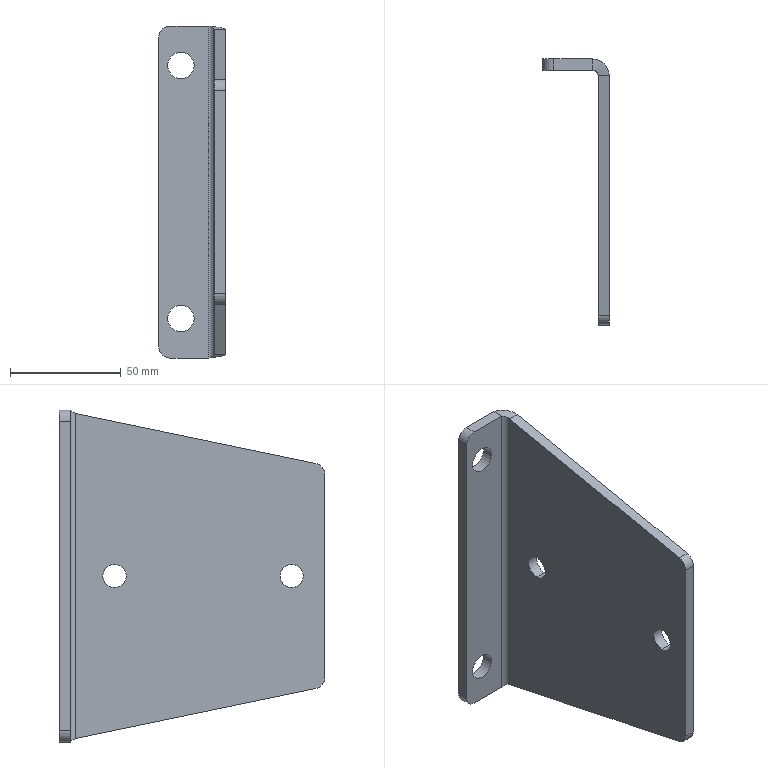Component | SolidWorks | JGS01-0001EndCorner-1 | 1 solid | 26 faces | box 30 x 120 x 150 mm | volume 90055 mm3 | cylinder 14 | plane 10 | spline 2 | commonest cylinder face diameters 10.5 x4 12 x4 10 x4 15 x1 5 x1 | material Plain Carbon Steel
STEP:
#1=COLOUR_RGB('',0.7922,0.8196,0.9333);
#2=FILL_AREA_STYLE_COLOUR('',#1);
#3=FILL_AREA_STYLE('',(#2));
#4=SURFACE_STYLE_FILL_AREA(#3);
#5=SURFACE_SIDE_STYLE('',(#4));
#6=SURFACE_STYLE_USAGE(.BOTH.,#5);
#7=PRESENTATION_STYLE_ASSIGNMENT((#6));
#8=CARTESIAN_POINT('',(-6.855,0.3688,13.707));
#9=VERTEX_POINT('',#8);
#10=CARTESIAN_POINT('',(-6.855,0.3688,13.293));
#11=VERTEX_POINT('',#10);
#12=CARTESIAN_POINT('',(-6.855,0.3688,13.5));
#13=DIRECTION('',(1.,0.,0.));
#14=DIRECTION('',(0.,0.,-1.));
#15=AXIS2_PLACEMENT_3D('',#12,#13,#14);
#16=CIRCLE('',#15,0.2067);
#17=EDGE_CURVE('',#9,#11,#16,.T.);
#18=ORIENTED_EDGE('',*,*,#17,.F.);
#19=CARTESIAN_POINT('',(-6.658,0.3688,13.707));
#20=VERTEX_POINT('',#19);
#21=CARTESIAN_POINT('',(-6.855,0.3688,13.707));
#22=DIRECTION('',(1.,0.,0.));
#23=VECTOR('',#22,39.37);
#24=LINE('',#21,#23);
#25=EDGE_CURVE('',#9,#20,#24,.T.);
#26=ORIENTED_EDGE('',*,*,#25,.T.);
#27=CARTESIAN_POINT('',(-6.658,0.3688,13.293));
#28=VERTEX_POINT('',#27);
#29=CARTESIAN_POINT('',(-6.658,0.3688,13.5));
#30=DIRECTION('',(1.,0.,0.));
#31=DIRECTION('',(0.,0.,-1.));
#32=AXIS2_PLACEMENT_3D('',#29,#30,#31);
#33=CIRCLE('',#32,0.2067);
#34=EDGE_CURVE('',#20,#28,#33,.T.);
#35=ORIENTED_EDGE('',*,*,#34,.T.);
#36=CARTESIAN_POINT('',(-6.855,0.3688,13.293));
#37=DIRECTION('',(1.,0.,0.));
#38=VECTOR('',#37,39.37);
#39=LINE('',#36,#38);
#40=EDGE_CURVE('',#11,#28,#39,.T.);
#41=ORIENTED_EDGE('',*,*,#40,.F.);
#42=EDGE_LOOP('',(#18,#26,#35,#41));
#43=FACE_OUTER_BOUND('',#42,.T.);
#44=CARTESIAN_POINT('',(-6.855,0.3688,13.5));
#45=DIRECTION('',(1.,0.,0.));
#46=DIRECTION('',(0.,0.,-1.));
#47=AXIS2_PLACEMENT_3D('',#44,#45,#46);
#48=CYLINDRICAL_SURFACE('',#47,0.2067);
#49=ADVANCED_FACE('',(#43),#48,.F.);
#50=CARTESIAN_POINT('',(-6.855,-2.781,13.707));
#51=VERTEX_POINT('',#50);
#52=CARTESIAN_POINT('',(-6.855,-2.781,13.293));
#53=VERTEX_POINT('',#52);
#54=CARTESIAN_POINT('',(-6.855,-2.781,13.5));
#55=DIRECTION('',(1.,0.,0.));
#56=DIRECTION('',(0.,0.,-1.));
#57=AXIS2_PLACEMENT_3D('',#54,#55,#56);
#58=CIRCLE('',#57,0.2067);
#59=EDGE_CURVE('',#51,#53,#58,.T.);
#60=ORIENTED_EDGE('',*,*,#59,.F.);
#61=CARTESIAN_POINT('',(-6.658,-2.781,13.707));
#62=VERTEX_POINT('',#61);
#63=CARTESIAN_POINT('',(-6.855,-2.781,13.707));
#64=DIRECTION('',(1.,0.,0.));
#65=VECTOR('',#64,39.37);
#66=LINE('',#63,#65);
#67=EDGE_CURVE('',#51,#62,#66,.T.);
#68=ORIENTED_EDGE('',*,*,#67,.T.);
#69=CARTESIAN_POINT('',(-6.658,-2.781,13.293));
#70=VERTEX_POINT('',#69);
#71=CARTESIAN_POINT('',(-6.658,-2.781,13.5));
#72=DIRECTION('',(1.,0.,0.));
#73=DIRECTION('',(0.,0.,-1.));
#74=AXIS2_PLACEMENT_3D('',#71,#72,#73);
#75=CIRCLE('',#74,0.2067);
#76=EDGE_CURVE('',#62,#70,#75,.T.);
#77=ORIENTED_EDGE('',*,*,#76,.T.);
#78=CARTESIAN_POINT('',(-6.855,-2.781,13.293));
#79=DIRECTION('',(1.,0.,0.));
#80=VECTOR('',#79,39.37);
#81=LINE('',#78,#80);
#82=EDGE_CURVE('',#53,#70,#81,.T.);
#83=ORIENTED_EDGE('',*,*,#82,.F.);
#84=EDGE_LOOP('',(#60,#68,#77,#83));
#85=FACE_OUTER_BOUND('',#84,.T.);
#86=CARTESIAN_POINT('',(-6.855,-2.781,13.5));
#87=DIRECTION('',(1.,0.,0.));
#88=DIRECTION('',(0.,0.,-1.));
#89=AXIS2_PLACEMENT_3D('',#86,#87,#88);
#90=CYLINDRICAL_SURFACE('',#89,0.2067);
#91=ADVANCED_FACE('',(#85),#90,.F.);
#92=CARTESIAN_POINT('',(-7.209,1.156,15.75));
#93=VERTEX_POINT('',#92);
#94=CARTESIAN_POINT('',(-7.682,1.156,15.75));
#95=VERTEX_POINT('',#94);
#96=CARTESIAN_POINT('',(-7.446,1.156,15.75));
#97=DIRECTION('',(0.,1.,0.));
#98=DIRECTION('',(-1.,0.,0.));
#99=AXIS2_PLACEMENT_3D('',#96,#97,#98);
#100=CIRCLE('',#99,0.2362);
#101=EDGE_CURVE('',#93,#95,#100,.T.);
#102=ORIENTED_EDGE('',*,*,#101,.F.);
#103=CARTESIAN_POINT('',(-7.209,1.353,15.75));
#104=VERTEX_POINT('',#103);
#105=CARTESIAN_POINT('',(-7.209,1.156,15.75));
#106=DIRECTION('',(0.,1.,0.));
#107=VECTOR('',#106,39.37);
#108=LINE('',#105,#107);
#109=EDGE_CURVE('',#93,#104,#108,.T.);
#110=ORIENTED_EDGE('',*,*,#109,.T.);
#111=CARTESIAN_POINT('',(-7.682,1.353,15.75));
#112=VERTEX_POINT('',#111);
#113=CARTESIAN_POINT('',(-7.446,1.353,15.75));
#114=DIRECTION('',(0.,1.,0.));
#115=DIRECTION('',(-1.,0.,0.));
#116=AXIS2_PLACEMENT_3D('',#113,#114,#115);
#117=CIRCLE('',#116,0.2362);
#118=EDGE_CURVE('',#104,#112,#117,.T.);
#119=ORIENTED_EDGE('',*,*,#118,.T.);
#120=CARTESIAN_POINT('',(-7.682,1.156,15.75));
#121=DIRECTION('',(0.,1.,0.));
#122=VECTOR('',#121,39.37);
#123=LINE('',#120,#122);
#124=EDGE_CURVE('',#95,#112,#123,.T.);
#125=ORIENTED_EDGE('',*,*,#124,.F.);
#126=EDGE_LOOP('',(#102,#110,#119,#125));
#127=FACE_OUTER_BOUND('',#126,.T.);
#128=CARTESIAN_POINT('',(-7.446,1.156,15.75));
#129=DIRECTION('',(0.,1.,0.));
#130=DIRECTION('',(-1.,0.,0.));
#131=AXIS2_PLACEMENT_3D('',#128,#129,#130);
#132=CYLINDRICAL_SURFACE('',#131,0.2362);
#133=ADVANCED_FACE('',(#127),#132,.F.);
#134=CARTESIAN_POINT('',(-7.209,1.156,11.25));
#135=VERTEX_POINT('',#134);
#136=CARTESIAN_POINT('',(-7.682,1.156,11.25));
#137=VERTEX_POINT('',#136);
#138=CARTESIAN_POINT('',(-7.446,1.156,11.25));
#139=DIRECTION('',(0.,1.,0.));
#140=DIRECTION('',(-1.,0.,0.));
#141=AXIS2_PLACEMENT_3D('',#138,#139,#140);
#142=CIRCLE('',#141,0.2362);
#143=EDGE_CURVE('',#135,#137,#142,.T.);
#144=ORIENTED_EDGE('',*,*,#143,.F.);
#145=CARTESIAN_POINT('',(-7.209,1.353,11.25));
#146=VERTEX_POINT('',#145);
#147=CARTESIAN_POINT('',(-7.209,1.156,11.25));
#148=DIRECTION('',(0.,1.,0.));
#149=VECTOR('',#148,39.37);
#150=LINE('',#147,#149);
#151=EDGE_CURVE('',#135,#146,#150,.T.);
#152=ORIENTED_EDGE('',*,*,#151,.T.);
#153=CARTESIAN_POINT('',(-7.682,1.353,11.25));
#154=VERTEX_POINT('',#153);
#155=CARTESIAN_POINT('',(-7.446,1.353,11.25));
#156=DIRECTION('',(0.,1.,0.));
#157=DIRECTION('',(-1.,0.,0.));
#158=AXIS2_PLACEMENT_3D('',#155,#156,#157);
#159=CIRCLE('',#158,0.2362);
#160=EDGE_CURVE('',#146,#154,#159,.T.);
#161=ORIENTED_EDGE('',*,*,#160,.T.);
#162=CARTESIAN_POINT('',(-7.682,1.156,11.25));
#163=DIRECTION('',(0.,1.,0.));
#164=VECTOR('',#163,39.37);
#165=LINE('',#162,#164);
#166=EDGE_CURVE('',#137,#154,#165,.T.);
#167=ORIENTED_EDGE('',*,*,#166,.F.);
#168=EDGE_LOOP('',(#144,#152,#161,#167));
#169=FACE_OUTER_BOUND('',#168,.T.);
#170=CARTESIAN_POINT('',(-7.446,1.156,11.25));
#171=DIRECTION('',(0.,1.,0.));
#172=DIRECTION('',(-1.,0.,0.));
#173=AXIS2_PLACEMENT_3D('',#170,#171,#172);
#174=CYLINDRICAL_SURFACE('',#173,0.2362);
#175=ADVANCED_FACE('',(#169),#174,.F.);
#176=CARTESIAN_POINT('',(-6.658,-3.215,11.499));
#177=VERTEX_POINT('',#176);
#178=CARTESIAN_POINT('',(-6.658,1.058,10.609));
#179=VERTEX_POINT('',#178);
#180=CARTESIAN_POINT('',(-6.658,-3.371,11.531));
#181=DIRECTION('',(0.,0.979,-0.204));
#182=VECTOR('',#181,39.37);
#183=LINE('',#180,#182);
#184=EDGE_CURVE('',#177,#179,#183,.T.);
#185=ORIENTED_EDGE('',*,*,#184,.F.);
#186=CARTESIAN_POINT('',(-6.855,-3.215,11.499));
#187=VERTEX_POINT('',#186);
#188=CARTESIAN_POINT('',(-6.855,-3.215,11.499));
#189=DIRECTION('',(-1.,0.,0.));
#190=VECTOR('',#189,39.37);
#191=LINE('',#188,#190);
#192=EDGE_CURVE('',#177,#187,#191,.T.);
#193=ORIENTED_EDGE('',*,*,#192,.T.);
#194=CARTESIAN_POINT('',(-6.855,1.058,10.609));
#195=VERTEX_POINT('',#194);
#196=CARTESIAN_POINT('',(-6.855,-3.371,11.531));
#197=DIRECTION('',(0.,0.979,-0.204));
#198=VECTOR('',#197,39.37);
#199=LINE('',#196,#198);
#200=EDGE_CURVE('',#187,#195,#199,.T.);
#201=ORIENTED_EDGE('',*,*,#200,.T.);
#202=CARTESIAN_POINT('',(-6.855,1.058,10.609));
#203=DIRECTION('',(1.,0.,0.));
#204=VECTOR('',#203,39.37);
#205=LINE('',#202,#204);
#206=EDGE_CURVE('',#195,#179,#205,.T.);
#207=ORIENTED_EDGE('',*,*,#206,.T.);
#208=EDGE_LOOP('',(#185,#193,#201,#207));
#209=FACE_OUTER_BOUND('',#208,.T.);
#210=CARTESIAN_POINT('',(-6.855,-3.371,11.531));
#211=DIRECTION('',(0.,-0.204,-0.979));
#212=DIRECTION('',(0.,0.979,-0.204));
#213=AXIS2_PLACEMENT_3D('',#210,#211,#212);
#214=PLANE('',#213);
#215=ADVANCED_FACE('',(#209),#214,.T.);
#216=CARTESIAN_POINT('',(-6.855,0.3688,13.5));
#217=DIRECTION('',(1.,0.,0.));
#218=DIRECTION('',(0.,0.,-1.));
#219=AXIS2_PLACEMENT_3D('',#216,#217,#218);
#220=CIRCLE('',#219,0.2067);
#221=EDGE_CURVE('',#11,#9,#220,.T.);
#222=ORIENTED_EDGE('',*,*,#221,.T.);
#223=ORIENTED_EDGE('',*,*,#17,.T.);
#224=EDGE_LOOP('',(#222,#223));
#225=FACE_BOUND('',#224,.T.);
#226=CARTESIAN_POINT('',(-6.855,-2.781,13.5));
#227=DIRECTION('',(1.,0.,0.));
#228=DIRECTION('',(0.,0.,-1.));
#229=AXIS2_PLACEMENT_3D('',#226,#227,#228);
#230=CIRCLE('',#229,0.2067);
#231=EDGE_CURVE('',#53,#51,#230,.T.);
#232=ORIENTED_EDGE('',*,*,#231,.T.);
#233=ORIENTED_EDGE('',*,*,#59,.T.);
#234=EDGE_LOOP('',(#232,#233));
#235=FACE_BOUND('',#234,.T.);
#236=CARTESIAN_POINT('',(-6.855,-3.371,15.308));
#237=VERTEX_POINT('',#236);
#238=CARTESIAN_POINT('',(-6.855,-3.371,11.692));
#239=VERTEX_POINT('',#238);
#240=CARTESIAN_POINT('',(-6.855,-3.371,15.469));
#241=DIRECTION('',(0.,0.,-1.));
#242=VECTOR('',#241,39.37);
#243=LINE('',#240,#242);
#244=EDGE_CURVE('',#237,#239,#243,.T.);
#245=ORIENTED_EDGE('',*,*,#244,.F.);
#246=CARTESIAN_POINT('',(-6.855,-3.215,15.501));
#247=VERTEX_POINT('',#246);
#248=CARTESIAN_POINT('',(-6.855,-3.175,15.308));
#249=DIRECTION('',(-1.,0.,0.));
#250=DIRECTION('',(0.,0.,-1.));
#251=AXIS2_PLACEMENT_3D('',#248,#249,#250);
#252=CIRCLE('',#251,0.1969);
#253=EDGE_CURVE('',#237,#247,#252,.T.);
#254=ORIENTED_EDGE('',*,*,#253,.T.);
#255=CARTESIAN_POINT('',(-6.855,1.058,16.391));
#256=VERTEX_POINT('',#255);
#257=CARTESIAN_POINT('',(-6.855,1.353,16.453));
#258=DIRECTION('',(0.,-0.979,-0.204));
#259=VECTOR('',#258,39.37);
#260=LINE('',#257,#259);
#261=EDGE_CURVE('',#256,#247,#260,.T.);
#262=ORIENTED_EDGE('',*,*,#261,.F.);
#263=CARTESIAN_POINT('',(-6.855,1.058,10.547));
#264=DIRECTION('',(0.,0.,1.));
#265=VECTOR('',#264,39.37);
#266=LINE('',#263,#265);
#267=EDGE_CURVE('',#195,#256,#266,.T.);
#268=ORIENTED_EDGE('',*,*,#267,.F.);
#269=ORIENTED_EDGE('',*,*,#200,.F.);
#270=CARTESIAN_POINT('',(-6.855,-3.175,11.692));
#271=DIRECTION('',(-1.,0.,0.));
#272=DIRECTION('',(0.,0.,-1.));
#273=AXIS2_PLACEMENT_3D('',#270,#271,#272);
#274=CIRCLE('',#273,0.1969);
#275=EDGE_CURVE('',#187,#239,#274,.T.);
#276=ORIENTED_EDGE('',*,*,#275,.T.);
#277=EDGE_LOOP('',(#245,#254,#262,#268,#269,#276));
#278=FACE_OUTER_BOUND('',#277,.T.);
#279=CARTESIAN_POINT('',(-6.855,-3.371,13.5));
#280=DIRECTION('',(1.,0.,0.));
#281=DIRECTION('',(0.,0.,-1.));
#282=AXIS2_PLACEMENT_3D('',#279,#280,#281);
#283=PLANE('',#282);
#284=ADVANCED_FACE('',(#225,#235,#278),#283,.F.);
#285=CARTESIAN_POINT('',(-6.658,0.3688,13.5));
#286=DIRECTION('',(1.,0.,0.));
#287=DIRECTION('',(0.,0.,-1.));
#288=AXIS2_PLACEMENT_3D('',#285,#286,#287);
#289=CIRCLE('',#288,0.2067);
#290=EDGE_CURVE('',#28,#20,#289,.T.);
#291=ORIENTED_EDGE('',*,*,#290,.F.);
#292=ORIENTED_EDGE('',*,*,#34,.F.);
#293=EDGE_LOOP('',(#291,#292));
#294=FACE_BOUND('',#293,.T.);
#295=CARTESIAN_POINT('',(-6.658,-2.781,13.5));
#296=DIRECTION('',(1.,0.,0.));
#297=DIRECTION('',(0.,0.,-1.));
#298=AXIS2_PLACEMENT_3D('',#295,#296,#297);
#299=CIRCLE('',#298,0.2067);
#300=EDGE_CURVE('',#70,#62,#299,.T.);
#301=ORIENTED_EDGE('',*,*,#300,.F.);
#302=ORIENTED_EDGE('',*,*,#76,.F.);
#303=EDGE_LOOP('',(#301,#302));
#304=FACE_BOUND('',#303,.T.);
#305=CARTESIAN_POINT('',(-6.658,1.058,16.391));
#306=VERTEX_POINT('',#305);
#307=CARTESIAN_POINT('',(-6.658,-3.215,15.501));
#308=VERTEX_POINT('',#307);
#309=CARTESIAN_POINT('',(-6.658,1.353,16.453));
#310=DIRECTION('',(0.,-0.979,-0.204));
#311=VECTOR('',#310,39.37);
#312=LINE('',#309,#311);
#313=EDGE_CURVE('',#306,#308,#312,.T.);
#314=ORIENTED_EDGE('',*,*,#313,.T.);
#315=CARTESIAN_POINT('',(-6.658,-3.371,15.308));
#316=VERTEX_POINT('',#315);
#317=CARTESIAN_POINT('',(-6.658,-3.175,15.308));
#318=DIRECTION('',(1.,0.,0.));
#319=DIRECTION('',(0.,0.,-1.));
#320=AXIS2_PLACEMENT_3D('',#317,#318,#319);
#321=CIRCLE('',#320,0.1969);
#322=EDGE_CURVE('',#308,#316,#321,.T.);
#323=ORIENTED_EDGE('',*,*,#322,.T.);
#324=CARTESIAN_POINT('',(-6.658,-3.371,11.692));
#325=VERTEX_POINT('',#324);
#326=CARTESIAN_POINT('',(-6.658,-3.371,15.469));
#327=DIRECTION('',(0.,0.,-1.));
#328=VECTOR('',#327,39.37);
#329=LINE('',#326,#328);
#330=EDGE_CURVE('',#316,#325,#329,.T.);
#331=ORIENTED_EDGE('',*,*,#330,.T.);
#332=CARTESIAN_POINT('',(-6.658,-3.175,11.692));
#333=DIRECTION('',(1.,0.,0.));
#334=DIRECTION('',(0.,0.,-1.));
#335=AXIS2_PLACEMENT_3D('',#332,#333,#334);
#336=CIRCLE('',#335,0.1969);
#337=EDGE_CURVE('',#325,#177,#336,.T.);
#338=ORIENTED_EDGE('',*,*,#337,.T.);
#339=ORIENTED_EDGE('',*,*,#184,.T.);
#340=CARTESIAN_POINT('',(-6.658,1.058,10.547));
#341=DIRECTION('',(0.,0.,1.));
#342=VECTOR('',#341,39.37);
#343=LINE('',#340,#342);
#344=EDGE_CURVE('',#179,#306,#343,.T.);
#345=ORIENTED_EDGE('',*,*,#344,.T.);
#346=EDGE_LOOP('',(#314,#323,#331,#338,#339,#345));
#347=FACE_OUTER_BOUND('',#346,.T.);
#348=CARTESIAN_POINT('',(-6.658,-3.371,13.5));
#349=DIRECTION('',(1.,0.,0.));
#350=DIRECTION('',(0.,0.,-1.));
#351=AXIS2_PLACEMENT_3D('',#348,#349,#350);
#352=PLANE('',#351);
#353=ADVANCED_FACE('',(#294,#304,#347),#352,.T.);
#354=ORIENTED_EDGE('',*,*,#261,.T.);
#355=CARTESIAN_POINT('',(-6.855,-3.215,15.501));
#356=DIRECTION('',(1.,0.,0.));
#357=VECTOR('',#356,39.37);
#358=LINE('',#355,#357);
#359=EDGE_CURVE('',#247,#308,#358,.T.);
#360=ORIENTED_EDGE('',*,*,#359,.T.);
#361=ORIENTED_EDGE('',*,*,#313,.F.);
#362=CARTESIAN_POINT('',(-6.855,1.058,16.391));
#363=DIRECTION('',(1.,0.,0.));
#364=VECTOR('',#363,39.37);
#365=LINE('',#362,#364);
#366=EDGE_CURVE('',#256,#306,#365,.T.);
#367=ORIENTED_EDGE('',*,*,#366,.F.);
#368=EDGE_LOOP('',(#354,#360,#361,#367));
#369=FACE_OUTER_BOUND('',#368,.T.);
#370=CARTESIAN_POINT('',(-6.855,1.353,16.453));
#371=DIRECTION('',(0.,-0.204,0.979));
#372=DIRECTION('',(0.,-0.979,-0.204));
#373=AXIS2_PLACEMENT_3D('',#370,#371,#372);
#374=PLANE('',#373);
#375=ADVANCED_FACE('',(#369),#374,.T.);
#376=ORIENTED_EDGE('',*,*,#330,.F.);
#377=CARTESIAN_POINT('',(-6.855,-3.371,15.308));
#378=DIRECTION('',(-1.,0.,0.));
#379=VECTOR('',#378,39.37);
#380=LINE('',#377,#379);
#381=EDGE_CURVE('',#316,#237,#380,.T.);
#382=ORIENTED_EDGE('',*,*,#381,.T.);
#383=ORIENTED_EDGE('',*,*,#244,.T.);
#384=CARTESIAN_POINT('',(-6.855,-3.371,11.692));
#385=DIRECTION('',(1.,0.,0.));
#386=VECTOR('',#385,39.37);
#387=LINE('',#384,#386);
#388=EDGE_CURVE('',#239,#325,#387,.T.);
#389=ORIENTED_EDGE('',*,*,#388,.T.);
#390=EDGE_LOOP('',(#376,#382,#383,#389));
#391=FACE_OUTER_BOUND('',#390,.T.);
#392=CARTESIAN_POINT('',(-6.855,-3.371,15.469));
#393=DIRECTION('',(0.,-1.,0.));
#394=DIRECTION('',(0.,0.,-1.));
#395=AXIS2_PLACEMENT_3D('',#392,#393,#394);
#396=PLANE('',#395);
#397=ADVANCED_FACE('',(#391),#396,.T.);
#398=CARTESIAN_POINT('',(-6.953,1.156,16.453));
#399=VERTEX_POINT('',#398);
#400=CARTESIAN_POINT('',(-6.953,1.353,16.453));
#401=VERTEX_POINT('',#400);
#402=CARTESIAN_POINT('',(-6.953,1.353,16.453));
#403=DIRECTION('',(0.,1.,0.));
#404=VECTOR('',#403,39.37);
#405=LINE('',#402,#404);
#406=EDGE_CURVE('',#399,#401,#405,.T.);
#407=ORIENTED_EDGE('',*,*,#406,.F.);
#408=CARTESIAN_POINT('',(-6.855,1.058,16.391));
#409=CARTESIAN_POINT('',(-6.855,1.064,16.394));
#410=CARTESIAN_POINT('',(-6.856,1.071,16.396));
#411=CARTESIAN_POINT('',(-6.858,1.083,16.401));
#412=CARTESIAN_POINT('',(-6.86,1.089,16.404));
#413=CARTESIAN_POINT('',(-6.865,1.101,16.409));
#414=CARTESIAN_POINT('',(-6.868,1.107,16.412));
#415=CARTESIAN_POINT('',(-6.875,1.118,16.417));
#416=CARTESIAN_POINT('',(-6.879,1.123,16.419));
#417=CARTESIAN_POINT('',(-6.888,1.132,16.425));
#418=CARTESIAN_POINT('',(-6.893,1.136,16.427));
#419=CARTESIAN_POINT('',(-6.904,1.143,16.432));
#420=CARTESIAN_POINT('',(-6.91,1.146,16.435));
#421=CARTESIAN_POINT('',(-6.922,1.151,16.44));
#422=CARTESIAN_POINT('',(-6.928,1.153,16.442));
#423=CARTESIAN_POINT('',(-6.94,1.156,16.448));
#424=CARTESIAN_POINT('',(-6.947,1.156,16.45));
#425=CARTESIAN_POINT('',(-6.953,1.156,16.453));
#426=B_SPLINE_CURVE_WITH_KNOTS('',3,(#408,#409,#410,#411,#412,#413,#414,#415,#416,#417,#418,#419,#420,#421,#422,#423,#424,#425),.UNSPECIFIED.,.F.,.F.,(4,2,2,2,2,2,2,2,4),(0.,0.0005255,0.001051,0.001576,0.002102,0.002627,0.003153,0.003678,0.004204),.UNSPECIFIED.);
#427=EDGE_CURVE('',#256,#399,#426,.T.);
#428=ORIENTED_EDGE('',*,*,#427,.F.);
#429=ORIENTED_EDGE('',*,*,#366,.T.);
#430=CARTESIAN_POINT('',(-6.658,1.058,16.391));
#431=CARTESIAN_POINT('',(-6.658,1.077,16.394));
#432=CARTESIAN_POINT('',(-6.66,1.096,16.396));
#433=CARTESIAN_POINT('',(-6.666,1.125,16.4));
#434=CARTESIAN_POINT('',(-6.668,1.134,16.401));
#435=CARTESIAN_POINT('',(-6.674,1.153,16.404));
#436=CARTESIAN_POINT('',(-6.677,1.162,16.405));
#437=CARTESIAN_POINT('',(-6.688,1.189,16.409));
#438=CARTESIAN_POINT('',(-6.697,1.206,16.412));
#439=CARTESIAN_POINT('',(-6.718,1.238,16.417));
#440=CARTESIAN_POINT('',(-6.731,1.253,16.419));
#441=CARTESIAN_POINT('',(-6.758,1.28,16.425));
#442=CARTESIAN_POINT('',(-6.773,1.292,16.427));
#443=CARTESIAN_POINT('',(-6.797,1.308,16.431));
#444=CARTESIAN_POINT('',(-6.806,1.314,16.432));
#445=CARTESIAN_POINT('',(-6.823,1.323,16.435));
#446=CARTESIAN_POINT('',(-6.831,1.327,16.436));
#447=CARTESIAN_POINT('',(-6.858,1.338,16.44));
#448=CARTESIAN_POINT('',(-6.876,1.343,16.442));
#449=CARTESIAN_POINT('',(-6.915,1.351,16.448));
#450=CARTESIAN_POINT('',(-6.934,1.353,16.45));
#451=CARTESIAN_POINT('',(-6.953,1.353,16.453));
#452=B_SPLINE_CURVE_WITH_KNOTS('',3,(#430,#431,#432,#433,#434,#435,#436,#437,#438,#439,#440,#441,#442,#443,#444,#445,#446,#447,#448,#449,#450,#451),.UNSPECIFIED.,.F.,.F.,(4,2,2,2,2,2,2,2,2,2,4),(0.,0.001477,0.002216,0.002955,0.004432,0.00591,0.007387,0.008126,0.008864,0.01034,0.01182),.UNSPECIFIED.);
#453=EDGE_CURVE('',#306,#401,#452,.T.);
#454=ORIENTED_EDGE('',*,*,#453,.T.);
#455=EDGE_LOOP('',(#407,#428,#429,#454));
#456=FACE_OUTER_BOUND('',#455,.T.);
#457=CARTESIAN_POINT('',(-6.656,1.058,16.391));
#458=CARTESIAN_POINT('',(-6.656,1.097,16.396));
#459=CARTESIAN_POINT('',(-6.664,1.136,16.401));
#460=CARTESIAN_POINT('',(-6.694,1.207,16.412));
#461=CARTESIAN_POINT('',(-6.716,1.24,16.417));
#462=CARTESIAN_POINT('',(-6.771,1.295,16.427));
#463=CARTESIAN_POINT('',(-6.804,1.317,16.432));
#464=CARTESIAN_POINT('',(-6.876,1.347,16.443));
#465=CARTESIAN_POINT('',(-6.914,1.355,16.448));
#466=CARTESIAN_POINT('',(-6.953,1.355,16.453));
#467=CARTESIAN_POINT('',(-6.658,1.058,16.391));
#468=CARTESIAN_POINT('',(-6.658,1.096,16.396));
#469=CARTESIAN_POINT('',(-6.666,1.135,16.401));
#470=CARTESIAN_POINT('',(-6.695,1.206,16.412));
#471=CARTESIAN_POINT('',(-6.717,1.239,16.417));
#472=CARTESIAN_POINT('',(-6.772,1.294,16.427));
#473=CARTESIAN_POINT('',(-6.805,1.316,16.432));
#474=CARTESIAN_POINT('',(-6.876,1.345,16.443));
#475=CARTESIAN_POINT('',(-6.915,1.353,16.448));
#476=CARTESIAN_POINT('',(-6.953,1.353,16.453));
#477=CARTESIAN_POINT('',(-6.855,1.058,16.391));
#478=CARTESIAN_POINT('',(-6.855,1.071,16.396));
#479=CARTESIAN_POINT('',(-6.858,1.084,16.401));
#480=CARTESIAN_POINT('',(-6.867,1.107,16.412));
#481=CARTESIAN_POINT('',(-6.875,1.118,16.417));
#482=CARTESIAN_POINT('',(-6.893,1.136,16.427));
#483=CARTESIAN_POINT('',(-6.904,1.144,16.432));
#484=CARTESIAN_POINT('',(-6.928,1.154,16.443));
#485=CARTESIAN_POINT('',(-6.94,1.156,16.448));
#486=CARTESIAN_POINT('',(-6.953,1.156,16.453));
#487=CARTESIAN_POINT('',(-6.857,1.058,16.391));
#488=CARTESIAN_POINT('',(-6.857,1.07,16.396));
#489=CARTESIAN_POINT('',(-6.859,1.083,16.401));
#490=CARTESIAN_POINT('',(-6.869,1.106,16.412));
#491=CARTESIAN_POINT('',(-6.876,1.117,16.417));
#492=CARTESIAN_POINT('',(-6.894,1.135,16.427));
#493=CARTESIAN_POINT('',(-6.905,1.142,16.432));
#494=CARTESIAN_POINT('',(-6.928,1.152,16.443));
#495=CARTESIAN_POINT('',(-6.941,1.154,16.448));
#496=CARTESIAN_POINT('',(-6.953,1.154,16.453));
#497=B_SPLINE_SURFACE_WITH_KNOTS('',1,3,((#457,#458,#459,#460,#461,#462,#463,#464,#465,#466),(#467,#468,#469,#470,#471,#472,#473,#474,#475,#476),(#477,#478,#479,#480,#481,#482,#483,#484,#485,#486),(#487,#488,#489,#490,#491,#492,#493,#494,#495,#496)),.UNSPECIFIED.,.F.,.F.,.F.,(2,1,1,2),(4,2,2,2,4),(-0.01,0.,1.,1.01),(0.,0.25,0.5,0.75,1.),.UNSPECIFIED.);
#498=ADVANCED_FACE('',(#456),#497,.F.);
#499=CARTESIAN_POINT('',(-6.953,1.156,10.547));
#500=VERTEX_POINT('',#499);
#501=CARTESIAN_POINT('',(-6.953,1.156,10.547));
#502=CARTESIAN_POINT('',(-6.947,1.156,10.55));
#503=CARTESIAN_POINT('',(-6.94,1.156,10.552));
#504=CARTESIAN_POINT('',(-6.928,1.153,10.557));
#505=CARTESIAN_POINT('',(-6.922,1.151,10.56));
#506=CARTESIAN_POINT('',(-6.91,1.146,10.565));
#507=CARTESIAN_POINT('',(-6.904,1.143,10.568));
#508=CARTESIAN_POINT('',(-6.893,1.136,10.573));
#509=CARTESIAN_POINT('',(-6.888,1.132,10.575));
#510=CARTESIAN_POINT('',(-6.879,1.123,10.581));
#511=CARTESIAN_POINT('',(-6.875,1.118,10.583));
#512=CARTESIAN_POINT('',(-6.868,1.107,10.588));
#513=CARTESIAN_POINT('',(-6.865,1.101,10.591));
#514=CARTESIAN_POINT('',(-6.86,1.09,10.596));
#515=CARTESIAN_POINT('',(-6.858,1.083,10.598));
#516=CARTESIAN_POINT('',(-6.856,1.071,10.604));
#517=CARTESIAN_POINT('',(-6.855,1.064,10.606));
#518=CARTESIAN_POINT('',(-6.855,1.058,10.609));
#519=B_SPLINE_CURVE_WITH_KNOTS('',3,(#501,#502,#503,#504,#505,#506,#507,#508,#509,#510,#511,#512,#513,#514,#515,#516,#517,#518),.UNSPECIFIED.,.F.,.F.,(4,2,2,2,2,2,2,2,4),(0.,0.0005255,0.001051,0.001576,0.002102,0.002627,0.003153,0.003678,0.004204),.UNSPECIFIED.);
#520=EDGE_CURVE('',#500,#195,#519,.T.);
#521=ORIENTED_EDGE('',*,*,#520,.F.);
#522=CARTESIAN_POINT('',(-6.953,1.353,10.547));
#523=VERTEX_POINT('',#522);
#524=CARTESIAN_POINT('',(-6.953,1.156,10.547));
#525=DIRECTION('',(0.,1.,0.));
#526=VECTOR('',#525,39.37);
#527=LINE('',#524,#526);
#528=EDGE_CURVE('',#500,#523,#527,.T.);
#529=ORIENTED_EDGE('',*,*,#528,.T.);
#530=CARTESIAN_POINT('',(-6.953,1.353,10.547));
#531=CARTESIAN_POINT('',(-6.934,1.353,10.55));
#532=CARTESIAN_POINT('',(-6.915,1.351,10.552));
#533=CARTESIAN_POINT('',(-6.886,1.345,10.556));
#534=CARTESIAN_POINT('',(-6.877,1.343,10.557));
#535=CARTESIAN_POINT('',(-6.859,1.338,10.56));
#536=CARTESIAN_POINT('',(-6.849,1.334,10.561));
#537=CARTESIAN_POINT('',(-6.823,1.323,10.565));
#538=CARTESIAN_POINT('',(-6.806,1.314,10.568));
#539=CARTESIAN_POINT('',(-6.773,1.293,10.573));
#540=CARTESIAN_POINT('',(-6.758,1.28,10.575));
#541=CARTESIAN_POINT('',(-6.731,1.253,10.581));
#542=CARTESIAN_POINT('',(-6.719,1.238,10.583));
#543=CARTESIAN_POINT('',(-6.703,1.214,10.587));
#544=CARTESIAN_POINT('',(-6.698,1.206,10.588));
#545=CARTESIAN_POINT('',(-6.688,1.189,10.591));
#546=CARTESIAN_POINT('',(-6.684,1.18,10.592));
#547=CARTESIAN_POINT('',(-6.673,1.153,10.596));
#548=CARTESIAN_POINT('',(-6.668,1.135,10.598));
#549=CARTESIAN_POINT('',(-6.66,1.097,10.604));
#550=CARTESIAN_POINT('',(-6.658,1.077,10.606));
#551=CARTESIAN_POINT('',(-6.658,1.058,10.609));
#552=B_SPLINE_CURVE_WITH_KNOTS('',3,(#530,#531,#532,#533,#534,#535,#536,#537,#538,#539,#540,#541,#542,#543,#544,#545,#546,#547,#548,#549,#550,#551),.UNSPECIFIED.,.F.,.F.,(4,2,2,2,2,2,2,2,2,2,4),(0.,0.001477,0.002216,0.002955,0.004432,0.00591,0.007387,0.008126,0.008864,0.01034,0.01182),.UNSPECIFIED.);
#553=EDGE_CURVE('',#523,#179,#552,.T.);
#554=ORIENTED_EDGE('',*,*,#553,.T.);
#555=ORIENTED_EDGE('',*,*,#206,.F.);
#556=EDGE_LOOP('',(#521,#529,#554,#555));
#557=FACE_OUTER_BOUND('',#556,.T.);
#558=CARTESIAN_POINT('',(-6.953,1.355,10.547));
#559=CARTESIAN_POINT('',(-6.914,1.355,10.552));
#560=CARTESIAN_POINT('',(-6.876,1.347,10.557));
#561=CARTESIAN_POINT('',(-6.804,1.317,10.568));
#562=CARTESIAN_POINT('',(-6.771,1.295,10.573));
#563=CARTESIAN_POINT('',(-6.716,1.24,10.583));
#564=CARTESIAN_POINT('',(-6.694,1.207,10.588));
#565=CARTESIAN_POINT('',(-6.664,1.136,10.599));
#566=CARTESIAN_POINT('',(-6.656,1.097,10.604));
#567=CARTESIAN_POINT('',(-6.656,1.058,10.609));
#568=CARTESIAN_POINT('',(-6.953,1.353,10.547));
#569=CARTESIAN_POINT('',(-6.915,1.353,10.552));
#570=CARTESIAN_POINT('',(-6.876,1.345,10.557));
#571=CARTESIAN_POINT('',(-6.805,1.316,10.568));
#572=CARTESIAN_POINT('',(-6.772,1.294,10.573));
#573=CARTESIAN_POINT('',(-6.717,1.239,10.583));
#574=CARTESIAN_POINT('',(-6.695,1.206,10.588));
#575=CARTESIAN_POINT('',(-6.666,1.135,10.599));
#576=CARTESIAN_POINT('',(-6.658,1.096,10.604));
#577=CARTESIAN_POINT('',(-6.658,1.058,10.609));
#578=CARTESIAN_POINT('',(-6.953,1.156,10.547));
#579=CARTESIAN_POINT('',(-6.94,1.156,10.552));
#580=CARTESIAN_POINT('',(-6.928,1.154,10.557));
#581=CARTESIAN_POINT('',(-6.904,1.144,10.568));
#582=CARTESIAN_POINT('',(-6.893,1.136,10.573));
#583=CARTESIAN_POINT('',(-6.875,1.118,10.583));
#584=CARTESIAN_POINT('',(-6.867,1.107,10.588));
#585=CARTESIAN_POINT('',(-6.858,1.084,10.599));
#586=CARTESIAN_POINT('',(-6.855,1.071,10.604));
#587=CARTESIAN_POINT('',(-6.855,1.058,10.609));
#588=CARTESIAN_POINT('',(-6.953,1.154,10.547));
#589=CARTESIAN_POINT('',(-6.941,1.154,10.552));
#590=CARTESIAN_POINT('',(-6.928,1.152,10.557));
#591=CARTESIAN_POINT('',(-6.905,1.142,10.568));
#592=CARTESIAN_POINT('',(-6.894,1.135,10.573));
#593=CARTESIAN_POINT('',(-6.876,1.117,10.583));
#594=CARTESIAN_POINT('',(-6.869,1.106,10.588));
#595=CARTESIAN_POINT('',(-6.859,1.083,10.599));
#596=CARTESIAN_POINT('',(-6.857,1.07,10.604));
#597=CARTESIAN_POINT('',(-6.857,1.058,10.609));
#598=B_SPLINE_SURFACE_WITH_KNOTS('',1,3,((#558,#559,#560,#561,#562,#563,#564,#565,#566,#567),(#568,#569,#570,#571,#572,#573,#574,#575,#576,#577),(#578,#579,#580,#581,#582,#583,#584,#585,#586,#587),(#588,#589,#590,#591,#592,#593,#594,#595,#596,#597)),.UNSPECIFIED.,.F.,.F.,.F.,(2,1,1,2),(4,2,2,2,4),(-0.01,0.,1.,1.01),(0.,0.25,0.5,0.75,1.),.UNSPECIFIED.);
#599=ADVANCED_FACE('',(#557),#598,.F.);
#600=ORIENTED_EDGE('',*,*,#344,.F.);
#601=ORIENTED_EDGE('',*,*,#553,.F.);
#602=CARTESIAN_POINT('',(-6.953,1.353,16.453));
#603=DIRECTION('',(0.,0.,1.));
#604=VECTOR('',#603,39.37);
#605=LINE('',#602,#604);
#606=EDGE_CURVE('',#523,#401,#605,.T.);
#607=ORIENTED_EDGE('',*,*,#606,.T.);
#608=ORIENTED_EDGE('',*,*,#453,.F.);
#609=EDGE_LOOP('',(#600,#601,#607,#608));
#610=FACE_OUTER_BOUND('',#609,.T.);
#611=CARTESIAN_POINT('',(-6.953,1.058,10.547));
#612=DIRECTION('',(0.,0.,-1.));
#613=DIRECTION('',(0.,1.,0.));
#614=AXIS2_PLACEMENT_3D('',#611,#612,#613);
#615=CYLINDRICAL_SURFACE('',#614,0.2953);
#616=ADVANCED_FACE('',(#610),#615,.T.);
#617=ORIENTED_EDGE('',*,*,#267,.T.);
#618=ORIENTED_EDGE('',*,*,#427,.T.);
#619=CARTESIAN_POINT('',(-6.953,1.156,16.453));
#620=DIRECTION('',(0.,0.,-1.));
#621=VECTOR('',#620,39.37);
#622=LINE('',#619,#621);
#623=EDGE_CURVE('',#399,#500,#622,.T.);
#624=ORIENTED_EDGE('',*,*,#623,.T.);
#625=ORIENTED_EDGE('',*,*,#520,.T.);
#626=EDGE_LOOP('',(#617,#618,#624,#625));
#627=FACE_OUTER_BOUND('',#626,.T.);
#628=CARTESIAN_POINT('',(-6.953,1.058,10.547));
#629=DIRECTION('',(0.,0.,-1.));
#630=DIRECTION('',(0.,1.,0.));
#631=AXIS2_PLACEMENT_3D('',#628,#629,#630);
#632=CYLINDRICAL_SURFACE('',#631,0.09843);
#633=ADVANCED_FACE('',(#627),#632,.F.);
#634=CARTESIAN_POINT('',(-7.642,1.156,10.547));
#635=VERTEX_POINT('',#634);
#636=CARTESIAN_POINT('',(-7.839,1.156,10.547));
#637=DIRECTION('',(-1.,0.,0.));
#638=VECTOR('',#637,39.37);
#639=LINE('',#636,#638);
#640=EDGE_CURVE('',#500,#635,#639,.T.);
#641=ORIENTED_EDGE('',*,*,#640,.T.);
#642=CARTESIAN_POINT('',(-7.642,1.353,10.547));
#643=VERTEX_POINT('',#642);
#644=CARTESIAN_POINT('',(-7.642,1.353,10.547));
#645=DIRECTION('',(0.,1.,0.));
#646=VECTOR('',#645,39.37);
#647=LINE('',#644,#646);
#648=EDGE_CURVE('',#635,#643,#647,.T.);
#649=ORIENTED_EDGE('',*,*,#648,.T.);
#650=CARTESIAN_POINT('',(-6.658,1.353,10.547));
#651=DIRECTION('',(-1.,0.,0.));
#652=VECTOR('',#651,39.37);
#653=LINE('',#650,#652);
#654=EDGE_CURVE('',#523,#643,#653,.T.);
#655=ORIENTED_EDGE('',*,*,#654,.F.);
#656=ORIENTED_EDGE('',*,*,#528,.F.);
#657=EDGE_LOOP('',(#641,#649,#655,#656));
#658=FACE_OUTER_BOUND('',#657,.T.);
#659=CARTESIAN_POINT('',(-7.839,1.353,10.547));
#660=DIRECTION('',(0.,0.,1.));
#661=DIRECTION('',(1.,0.,0.));
#662=AXIS2_PLACEMENT_3D('',#659,#660,#661);
#663=PLANE('',#662);
#664=ADVANCED_FACE('',(#658),#663,.F.);
#665=CARTESIAN_POINT('',(-7.642,1.353,16.453));
#666=VERTEX_POINT('',#665);
#667=CARTESIAN_POINT('',(-6.658,1.353,16.453));
#668=DIRECTION('',(1.,-0.,0.));
#669=VECTOR('',#668,39.37);
#670=LINE('',#667,#669);
#671=EDGE_CURVE('',#666,#401,#670,.T.);
#672=ORIENTED_EDGE('',*,*,#671,.F.);
#673=CARTESIAN_POINT('',(-7.642,1.156,16.453));
#674=VERTEX_POINT('',#673);
#675=CARTESIAN_POINT('',(-7.642,1.353,16.453));
#676=DIRECTION('',(-0.,-1.,0.));
#677=VECTOR('',#676,39.37);
#678=LINE('',#675,#677);
#679=EDGE_CURVE('',#666,#674,#678,.T.);
#680=ORIENTED_EDGE('',*,*,#679,.T.);
#681=CARTESIAN_POINT('',(-6.855,1.156,16.453));
#682=DIRECTION('',(1.,-0.,0.));
#683=VECTOR('',#682,39.37);
#684=LINE('',#681,#683);
#685=EDGE_CURVE('',#674,#399,#684,.T.);
#686=ORIENTED_EDGE('',*,*,#685,.T.);
#687=ORIENTED_EDGE('',*,*,#406,.T.);
#688=EDGE_LOOP('',(#672,#680,#686,#687));
#689=FACE_OUTER_BOUND('',#688,.T.);
#690=CARTESIAN_POINT('',(-6.855,1.353,16.453));
#691=DIRECTION('',(0.,0.,-1.));
#692=DIRECTION('',(-1.,0.,0.));
#693=AXIS2_PLACEMENT_3D('',#690,#691,#692);
#694=PLANE('',#693);
#695=ADVANCED_FACE('',(#689),#694,.F.);
#696=CARTESIAN_POINT('',(-7.446,1.353,15.75));
#697=DIRECTION('',(0.,1.,0.));
#698=DIRECTION('',(-1.,0.,0.));
#699=AXIS2_PLACEMENT_3D('',#696,#697,#698);
#700=CIRCLE('',#699,0.2362);
#701=EDGE_CURVE('',#112,#104,#700,.T.);
#702=ORIENTED_EDGE('',*,*,#701,.F.);
#703=ORIENTED_EDGE('',*,*,#118,.F.);
#704=EDGE_LOOP('',(#702,#703));
#705=FACE_BOUND('',#704,.T.);
#706=CARTESIAN_POINT('',(-7.446,1.353,11.25));
#707=DIRECTION('',(0.,1.,0.));
#708=DIRECTION('',(-1.,0.,0.));
#709=AXIS2_PLACEMENT_3D('',#706,#707,#708);
#710=CIRCLE('',#709,0.2362);
#711=EDGE_CURVE('',#154,#146,#710,.T.);
#712=ORIENTED_EDGE('',*,*,#711,.F.);
#713=ORIENTED_EDGE('',*,*,#160,.F.);
#714=EDGE_LOOP('',(#712,#713));
#715=FACE_BOUND('',#714,.T.);
#716=ORIENTED_EDGE('',*,*,#654,.T.);
#717=CARTESIAN_POINT('',(-7.839,1.353,10.744));
#718=VERTEX_POINT('',#717);
#719=CARTESIAN_POINT('',(-7.642,1.353,10.744));
#720=DIRECTION('',(0.,1.,0.));
#721=DIRECTION('',(1.,-0.,0.));
#722=AXIS2_PLACEMENT_3D('',#719,#720,#721);
#723=CIRCLE('',#722,0.1969);
#724=EDGE_CURVE('',#643,#718,#723,.T.);
#725=ORIENTED_EDGE('',*,*,#724,.T.);
#726=CARTESIAN_POINT('',(-7.839,1.353,16.256));
#727=VERTEX_POINT('',#726);
#728=CARTESIAN_POINT('',(-7.839,1.353,13.5));
#729=DIRECTION('',(0.,0.,1.));
#730=VECTOR('',#729,39.37);
#731=LINE('',#728,#730);
#732=EDGE_CURVE('',#718,#727,#731,.T.);
#733=ORIENTED_EDGE('',*,*,#732,.T.);
#734=CARTESIAN_POINT('',(-7.642,1.353,16.256));
#735=DIRECTION('',(0.,1.,0.));
#736=DIRECTION('',(1.,-0.,0.));
#737=AXIS2_PLACEMENT_3D('',#734,#735,#736);
#738=CIRCLE('',#737,0.1969);
#739=EDGE_CURVE('',#727,#666,#738,.T.);
#740=ORIENTED_EDGE('',*,*,#739,.T.);
#741=ORIENTED_EDGE('',*,*,#671,.T.);
#742=ORIENTED_EDGE('',*,*,#606,.F.);
#743=EDGE_LOOP('',(#716,#725,#733,#740,#741,#742));
#744=FACE_OUTER_BOUND('',#743,.T.);
#745=CARTESIAN_POINT('',(-6.658,1.353,13.5));
#746=DIRECTION('',(-0.,-1.,0.));
#747=DIRECTION('',(1.,-0.,0.));
#748=AXIS2_PLACEMENT_3D('',#745,#746,#747);
#749=PLANE('',#748);
#750=ADVANCED_FACE('',(#705,#715,#744),#749,.F.);
#751=CARTESIAN_POINT('',(-7.446,1.156,15.75));
#752=DIRECTION('',(0.,1.,0.));
#753=DIRECTION('',(-1.,0.,0.));
#754=AXIS2_PLACEMENT_3D('',#751,#752,#753);
#755=CIRCLE('',#754,0.2362);
#756=EDGE_CURVE('',#95,#93,#755,.T.);
#757=ORIENTED_EDGE('',*,*,#756,.T.);
#758=ORIENTED_EDGE('',*,*,#101,.T.);
#759=EDGE_LOOP('',(#757,#758));
#760=FACE_BOUND('',#759,.T.);
#761=CARTESIAN_POINT('',(-7.446,1.156,11.25));
#762=DIRECTION('',(0.,1.,0.));
#763=DIRECTION('',(-1.,0.,0.));
#764=AXIS2_PLACEMENT_3D('',#761,#762,#763);
#765=CIRCLE('',#764,0.2362);
#766=EDGE_CURVE('',#137,#135,#765,.T.);
#767=ORIENTED_EDGE('',*,*,#766,.T.);
#768=ORIENTED_EDGE('',*,*,#143,.T.);
#769=EDGE_LOOP('',(#767,#768));
#770=FACE_BOUND('',#769,.T.);
#771=CARTESIAN_POINT('',(-7.839,1.156,10.744));
#772=VERTEX_POINT('',#771);
#773=CARTESIAN_POINT('',(-7.839,1.156,16.256));
#774=VERTEX_POINT('',#773);
#775=CARTESIAN_POINT('',(-7.839,1.156,16.453));
#776=DIRECTION('',(0.,0.,1.));
#777=VECTOR('',#776,39.37);
#778=LINE('',#775,#777);
#779=EDGE_CURVE('',#772,#774,#778,.T.);
#780=ORIENTED_EDGE('',*,*,#779,.F.);
#781=CARTESIAN_POINT('',(-7.642,1.156,10.744));
#782=DIRECTION('',(-0.,-1.,0.));
#783=DIRECTION('',(1.,-0.,0.));
#784=AXIS2_PLACEMENT_3D('',#781,#782,#783);
#785=CIRCLE('',#784,0.1969);
#786=EDGE_CURVE('',#772,#635,#785,.T.);
#787=ORIENTED_EDGE('',*,*,#786,.T.);
#788=ORIENTED_EDGE('',*,*,#640,.F.);
#789=ORIENTED_EDGE('',*,*,#623,.F.);
#790=ORIENTED_EDGE('',*,*,#685,.F.);
#791=CARTESIAN_POINT('',(-7.642,1.156,16.256));
#792=DIRECTION('',(-0.,-1.,0.));
#793=DIRECTION('',(1.,-0.,0.));
#794=AXIS2_PLACEMENT_3D('',#791,#792,#793);
#795=CIRCLE('',#794,0.1969);
#796=EDGE_CURVE('',#674,#774,#795,.T.);
#797=ORIENTED_EDGE('',*,*,#796,.T.);
#798=EDGE_LOOP('',(#780,#787,#788,#789,#790,#797));
#799=FACE_OUTER_BOUND('',#798,.T.);
#800=CARTESIAN_POINT('',(-6.658,1.156,13.5));
#801=DIRECTION('',(-0.,-1.,0.));
#802=DIRECTION('',(1.,-0.,0.));
#803=AXIS2_PLACEMENT_3D('',#800,#801,#802);
#804=PLANE('',#803);
#805=ADVANCED_FACE('',(#760,#770,#799),#804,.T.);
#806=ORIENTED_EDGE('',*,*,#732,.F.);
#807=CARTESIAN_POINT('',(-7.839,1.353,10.744));
#808=DIRECTION('',(-0.,-1.,0.));
#809=VECTOR('',#808,39.37);
#810=LINE('',#807,#809);
#811=EDGE_CURVE('',#718,#772,#810,.T.);
#812=ORIENTED_EDGE('',*,*,#811,.T.);
#813=ORIENTED_EDGE('',*,*,#779,.T.);
#814=CARTESIAN_POINT('',(-7.839,1.353,16.256));
#815=DIRECTION('',(0.,1.,0.));
#816=VECTOR('',#815,39.37);
#817=LINE('',#814,#816);
#818=EDGE_CURVE('',#774,#727,#817,.T.);
#819=ORIENTED_EDGE('',*,*,#818,.T.);
#820=EDGE_LOOP('',(#806,#812,#813,#819));
#821=FACE_OUTER_BOUND('',#820,.T.);
#822=CARTESIAN_POINT('',(-7.839,1.353,16.453));
#823=DIRECTION('',(1.,-0.,0.));
#824=DIRECTION('',(0.,1.,0.));
#825=AXIS2_PLACEMENT_3D('',#822,#823,#824);
#826=PLANE('',#825);
#827=ADVANCED_FACE('',(#821),#826,.F.);
#828=ORIENTED_EDGE('',*,*,#724,.F.);
#829=ORIENTED_EDGE('',*,*,#648,.F.);
#830=ORIENTED_EDGE('',*,*,#786,.F.);
#831=ORIENTED_EDGE('',*,*,#811,.F.);
#832=EDGE_LOOP('',(#828,#829,#830,#831));
#833=FACE_OUTER_BOUND('',#832,.T.);
#834=CARTESIAN_POINT('',(-7.642,1.353,10.744));
#835=DIRECTION('',(-0.,-1.,0.));
#836=DIRECTION('',(1.,-0.,0.));
#837=AXIS2_PLACEMENT_3D('',#834,#835,#836);
#838=CYLINDRICAL_SURFACE('',#837,0.1969);
#839=ADVANCED_FACE('',(#833),#838,.T.);
#840=ORIENTED_EDGE('',*,*,#739,.F.);
#841=ORIENTED_EDGE('',*,*,#818,.F.);
#842=ORIENTED_EDGE('',*,*,#796,.F.);
#843=ORIENTED_EDGE('',*,*,#679,.F.);
#844=EDGE_LOOP('',(#840,#841,#842,#843));
#845=FACE_OUTER_BOUND('',#844,.T.);
#846=CARTESIAN_POINT('',(-7.642,1.353,16.256));
#847=DIRECTION('',(-0.,-1.,0.));
#848=DIRECTION('',(1.,-0.,0.));
#849=AXIS2_PLACEMENT_3D('',#846,#847,#848);
#850=CYLINDRICAL_SURFACE('',#849,0.1969);
#851=ADVANCED_FACE('',(#845),#850,.T.);
#852=ORIENTED_EDGE('',*,*,#253,.F.);
#853=ORIENTED_EDGE('',*,*,#381,.F.);
#854=ORIENTED_EDGE('',*,*,#322,.F.);
#855=ORIENTED_EDGE('',*,*,#359,.F.);
#856=EDGE_LOOP('',(#852,#853,#854,#855));
#857=FACE_OUTER_BOUND('',#856,.T.);
#858=CARTESIAN_POINT('',(-6.855,-3.175,15.308));
#859=DIRECTION('',(1.,0.,0.));
#860=DIRECTION('',(0.,0.,-1.));
#861=AXIS2_PLACEMENT_3D('',#858,#859,#860);
#862=CYLINDRICAL_SURFACE('',#861,0.1969);
#863=ADVANCED_FACE('',(#857),#862,.T.);
#864=ORIENTED_EDGE('',*,*,#275,.F.);
#865=ORIENTED_EDGE('',*,*,#192,.F.);
#866=ORIENTED_EDGE('',*,*,#337,.F.);
#867=ORIENTED_EDGE('',*,*,#388,.F.);
#868=EDGE_LOOP('',(#864,#865,#866,#867));
#869=FACE_OUTER_BOUND('',#868,.T.);
#870=CARTESIAN_POINT('',(-6.855,-3.175,11.692));
#871=DIRECTION('',(1.,0.,0.));
#872=DIRECTION('',(0.,0.,-1.));
#873=AXIS2_PLACEMENT_3D('',#870,#871,#872);
#874=CYLINDRICAL_SURFACE('',#873,0.1969);
#875=ADVANCED_FACE('',(#869),#874,.T.);
#876=ORIENTED_EDGE('',*,*,#151,.F.);
#877=ORIENTED_EDGE('',*,*,#766,.F.);
#878=ORIENTED_EDGE('',*,*,#166,.T.);
#879=ORIENTED_EDGE('',*,*,#711,.T.);
#880=EDGE_LOOP('',(#876,#877,#878,#879));
#881=FACE_OUTER_BOUND('',#880,.T.);
#882=CARTESIAN_POINT('',(-7.446,1.156,11.25));
#883=DIRECTION('',(0.,1.,0.));
#884=DIRECTION('',(-1.,0.,0.));
#885=AXIS2_PLACEMENT_3D('',#882,#883,#884);
#886=CYLINDRICAL_SURFACE('',#885,0.2362);
#887=ADVANCED_FACE('',(#881),#886,.F.);
#888=ORIENTED_EDGE('',*,*,#109,.F.);
#889=ORIENTED_EDGE('',*,*,#756,.F.);
#890=ORIENTED_EDGE('',*,*,#124,.T.);
#891=ORIENTED_EDGE('',*,*,#701,.T.);
#892=EDGE_LOOP('',(#888,#889,#890,#891));
#893=FACE_OUTER_BOUND('',#892,.T.);
#894=CARTESIAN_POINT('',(-7.446,1.156,15.75));
#895=DIRECTION('',(0.,1.,0.));
#896=DIRECTION('',(-1.,0.,0.));
#897=AXIS2_PLACEMENT_3D('',#894,#895,#896);
#898=CYLINDRICAL_SURFACE('',#897,0.2362);
#899=ADVANCED_FACE('',(#893),#898,.F.);
#900=ORIENTED_EDGE('',*,*,#67,.F.);
#901=ORIENTED_EDGE('',*,*,#231,.F.);
#902=ORIENTED_EDGE('',*,*,#82,.T.);
#903=ORIENTED_EDGE('',*,*,#300,.T.);
#904=EDGE_LOOP('',(#900,#901,#902,#903));
#905=FACE_OUTER_BOUND('',#904,.T.);
#906=CARTESIAN_POINT('',(-6.855,-2.781,13.5));
#907=DIRECTION('',(1.,0.,0.));
#908=DIRECTION('',(0.,0.,-1.));
#909=AXIS2_PLACEMENT_3D('',#906,#907,#908);
#910=CYLINDRICAL_SURFACE('',#909,0.2067);
#911=ADVANCED_FACE('',(#905),#910,.F.);
#912=ORIENTED_EDGE('',*,*,#25,.F.);
#913=ORIENTED_EDGE('',*,*,#221,.F.);
#914=ORIENTED_EDGE('',*,*,#40,.T.);
#915=ORIENTED_EDGE('',*,*,#290,.T.);
#916=EDGE_LOOP('',(#912,#913,#914,#915));
#917=FACE_OUTER_BOUND('',#916,.T.);
#918=CARTESIAN_POINT('',(-6.855,0.3688,13.5));
#919=DIRECTION('',(1.,0.,0.));
#920=DIRECTION('',(0.,0.,-1.));
#921=AXIS2_PLACEMENT_3D('',#918,#919,#920);
#922=CYLINDRICAL_SURFACE('',#921,0.2067);
#923=ADVANCED_FACE('',(#917),#922,.F.);
#924=CLOSED_SHELL('',(#49,#91,#133,#175,#215,#284,#353,#375,#397,#498,#599,#616,#633,#664,#695,#750,#805,#827,#839,#851,#863,#875,#887,#899,#911,#923));
#925=MANIFOLD_SOLID_BREP('',#924);
#926=STYLED_ITEM('',(#7),#925);
#927=PRESENTATION_LAYER_ASSIGNMENT('','',(#926));
#928=CARTESIAN_POINT('',(0.,0.,0.));
#929=DIRECTION('',(0.,0.,1.));
#930=DIRECTION('',(1.,0.,0.));
#931=AXIS2_PLACEMENT_3D('',#928,#929,#930);
#932=(LENGTH_UNIT()NAMED_UNIT(*)SI_UNIT($,.METRE.));
#933=LENGTH_MEASURE_WITH_UNIT(LENGTH_MEASURE(0.0254),#932);
#934=DIMENSIONAL_EXPONENTS(1.,0.,0.,0.,0.,0.,0.);
#935=(CONVERSION_BASED_UNIT('',#933)LENGTH_UNIT()NAMED_UNIT(#934));
#936=UNCERTAINTY_MEASURE_WITH_UNIT(LENGTH_MEASURE(0.00001),#935,'','');
#937=(NAMED_UNIT(*)PLANE_ANGLE_UNIT()SI_UNIT($,.RADIAN.));
#938=(NAMED_UNIT(*)SI_UNIT($,.STERADIAN.)SOLID_ANGLE_UNIT());
#939=(GEOMETRIC_REPRESENTATION_CONTEXT(3)GLOBAL_UNCERTAINTY_ASSIGNED_CONTEXT((#936))GLOBAL_UNIT_ASSIGNED_CONTEXT((#935,#937,#938))REPRESENTATION_CONTEXT('',''));
#940=ADVANCED_BREP_SHAPE_REPRESENTATION('',(#925,#931),#939);
#941=(LENGTH_UNIT()NAMED_UNIT(*)SI_UNIT($,.METRE.));
#942=LENGTH_MEASURE_WITH_UNIT(LENGTH_MEASURE(0.0254),#941);
#943=DIMENSIONAL_EXPONENTS(1.,0.,0.,0.,0.,0.,0.);
#944=(CONVERSION_BASED_UNIT('',#942)LENGTH_UNIT()NAMED_UNIT(#943));
#945=UNCERTAINTY_MEASURE_WITH_UNIT(LENGTH_MEASURE(0.00001),#944,'','');
#946=(NAMED_UNIT(*)PLANE_ANGLE_UNIT()SI_UNIT($,.RADIAN.));
#947=(NAMED_UNIT(*)SI_UNIT($,.STERADIAN.)SOLID_ANGLE_UNIT());
#948=(GEOMETRIC_REPRESENTATION_CONTEXT(3)GLOBAL_UNCERTAINTY_ASSIGNED_CONTEXT((#945))GLOBAL_UNIT_ASSIGNED_CONTEXT((#944,#946,#947))REPRESENTATION_CONTEXT('',''));
#949=MECHANICAL_DESIGN_GEOMETRIC_PRESENTATION_REPRESENTATION('',(#926),#948);